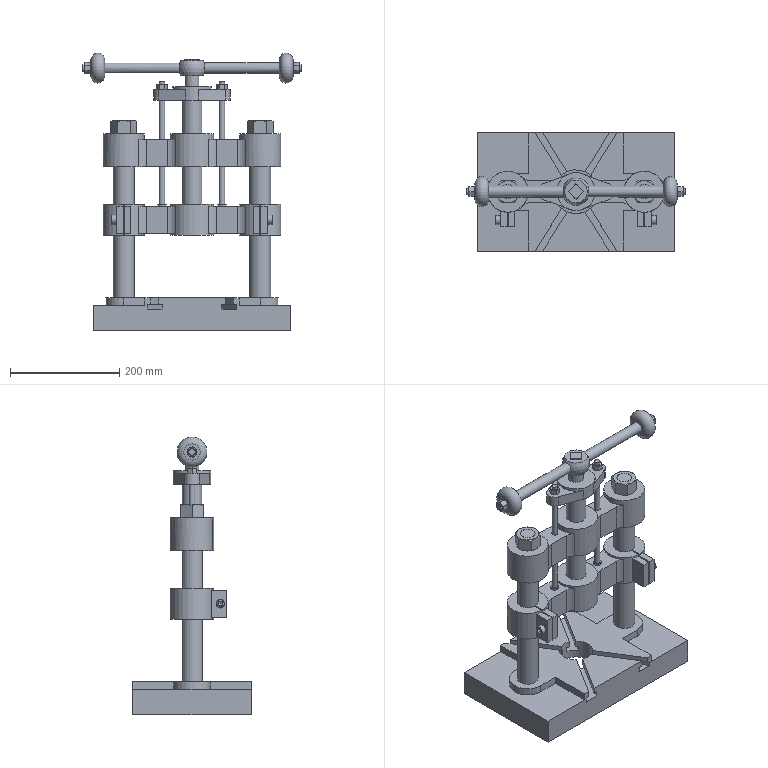Assembly | NX | mm | 23 component files | 23 solids | 474 faces | box 400 x 217 x 509 mm | volume 5898683 mm3 | plane 257 | cone 125 | cylinder 83 | torus 8 | sphere 1 | commonest cylinder face diameters 40 x16 27 x11 10 x6 9.732 x6 12 x4 75 x4 10.5 x4 11 x3
Bill of materials:
unnamed part 1 | 1 |  | Straight bar with a rounded central hub. The hub has a square through-opening, and two coaxial arms run out from it, each stepping down to a smaller diameter at its outer end.
GB-T41-2000,M27x3 | 4 |  | Hexagonal prism with a plain cylindrical through-bore along its axis and chamfered corners on both end faces; shaped like a hex nut.
unnamed part 2 | 1 |  | Stepped cylindrical shaft: a long main diameter, a shorter reduced-diameter step, and a flat-sided, rectangular-section tang at one end.
unnamed part 3 | 2 |  | Stepped cylindrical pin: a larger-diameter middle section with a smaller, coaxial diameter at each end. One end section is noticeably longer than the other.
GB-T41-2000,M12x1.75 | 2 |  | Hexagonal prism with a plain cylindrical through-bore along its axis and chamfered corners on both ends; looks like a hex nut, possibly slightly thicker relative to its width than the other two parts.
unnamed part 4 | 1 |  | Elongated plate-like body with three circular bosses in a row joined by thinner webs. The two end bosses are split by slots and have rectangular clamp-style ears with cross holes. The central boss has a bore, and each web has a small hole.
GB-T70.1-2000,M10x25 | 2 |  | Hexagon Socket Head Cap Screw, GB-T 70.1-2000,M10x25
unnamed part 5 | 1 |  | Two-lobed, diamond-shaped flange plate with a raised circular boss in the centre, a central through-bore, and a smaller through-hole in each rounded lobe.
unnamed part 6 | 1 |  | Rectangular block with shallow recessed features on its top face: a central circular recess, thin narrow channels radiating outward in roughly an X pattern, and two offset holes inside curved pocket outlines. The bottom view shows three through-holes in a row.
unnamed part 7 | 2 |  | Torus-like ring with a rounded outer profile and a small central through-hole.
unnamed part 8 | 2 |  | Plain, slender, straight cylindrical rod of uniform diameter with flat ends.
unnamed part 9 | 1 |  | Elongated body with three cylindrical bosses in a row joined by lower, thinner webs. Each boss has a through-bore, and each web has a small through-hole.
GB-T41-2000,M10x1.5 | 2 |  | Hexagonal prism with a plain cylindrical through-bore and chamfered corners on both end faces; nearly the same as unnamed part, but the bore looks a little smaller compared with the hex size.
GB-T70.1-2000,M10x30 | 1 |  | Hexagon Socket Head Cap Screw, GB-T 70.1-2000,M10x30
Mates:
1. fix | base 1 component
2. concentric | support_post 2 edge | base 1 arc
3. concentric | support_post 1 edge | base 1 arc
4. touch align | press_plate 1 face | support_post 2 face
5. touch align | press_plate 1 face | support_post 1 face
6. concentric | top_cover 1 edge | support_post 2 edge
7. concentric | screw_rod 1 edge | press_plate 1 edge
8. concentric | stud 2 arc | press_plate 1 arc
9. concentric | stud 1 arc | press_plate 1 arc
10. concentric | fixed_plate 1 edge | screw_rod 1 arc
11. concentric | stud 2 arc | fixed_plate 1 edge
12. concentric | grip 1 edge | screw_rod 1 edge
13. concentric | handle 2 edge | grip 1 edge
14. concentric | handle 1 edge | grip 1 edge
15. concentric | nut_M12 2 edge | handle 2 edge
16. concentric | nut_M27 1 edge | base 1 arc
17. concentric | nut_M27 2 edge | base 1 arc
18. concentric | nut_M27 3 edge | top_cover 1 edge
19. concentric | nut_M27 4 edge | top_cover 1 edge
20. concentric | nut_M10 2 edge | fixed_plate 1 edge
21. concentric | nut_M10 1 edge | fixed_plate 1 edge
22. concentric | nut_M12 1 edge | handle 1 edge